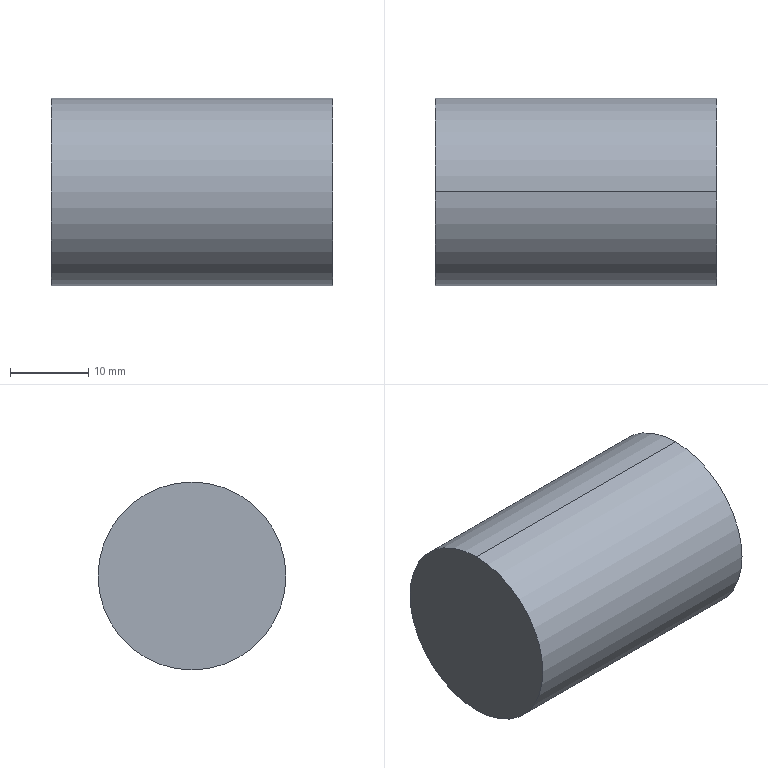Component | SolidWorks | PushRodCylinder-1 | 1 solid | 7 faces | box 36 x 24 x 24 mm | volume 15281 mm3 | cylinder 4 | plane 3 | commonest cylinder face diameters 8 x2 24 x2
build123d program:
from build123d import *

# Parameters (mm, degrees)
SKETCH1_R           = 12
BOSS_EXTRUDE1_DEPTH = 36
SKETCH2_R           = 4
CUT_EXTRUDE1_DEPTH  = 20


with BuildPart() as part:
    # Sketch1 → Boss-Extrude1 (new body)
    with BuildSketch(Plane.XY):
        Circle(SKETCH1_R)
    extrude(amount=BOSS_EXTRUDE1_DEPTH)

    # Sketch2 → Cut-Extrude1 (cut)
    with BuildSketch(Plane(origin=(0, 0, 0), x_dir=(-1, 0, 0), z_dir=(0, 0, -1))):
        Circle(SKETCH2_R)
    extrude(amount=-CUT_EXTRUDE1_DEPTH, mode=Mode.SUBTRACT)


solid = part.part

# Placed as in the assembly
solid = solid.moved(Location((-183.5, 220, -10), (0, -90, 0)))
STEP:
#1=COLOUR_RGB('',0.7922,0.8196,0.9333);
#2=FILL_AREA_STYLE_COLOUR('',#1);
#3=FILL_AREA_STYLE('',(#2));
#4=SURFACE_STYLE_FILL_AREA(#3);
#5=SURFACE_SIDE_STYLE('',(#4));
#6=SURFACE_STYLE_USAGE(.BOTH.,#5);
#7=PRESENTATION_STYLE_ASSIGNMENT((#6));
#8=CARTESIAN_POINT('',(-8.012,8.661,-0.2362));
#9=VERTEX_POINT('',#8);
#10=CARTESIAN_POINT('',(-8.012,8.661,-0.5512));
#11=VERTEX_POINT('',#10);
#12=CARTESIAN_POINT('',(-8.012,8.661,-0.3937));
#13=DIRECTION('',(1.,0.,0.));
#14=DIRECTION('',(0.,0.,-1.));
#15=AXIS2_PLACEMENT_3D('',#12,#13,#14);
#16=CIRCLE('',#15,0.1575);
#17=EDGE_CURVE('',#9,#11,#16,.T.);
#18=ORIENTED_EDGE('',*,*,#17,.F.);
#19=CARTESIAN_POINT('',(-7.224,8.661,-0.2362));
#20=VERTEX_POINT('',#19);
#21=CARTESIAN_POINT('',(-8.012,8.661,-0.2362));
#22=DIRECTION('',(1.,0.,0.));
#23=VECTOR('',#22,39.37);
#24=LINE('',#21,#23);
#25=EDGE_CURVE('',#9,#20,#24,.T.);
#26=ORIENTED_EDGE('',*,*,#25,.T.);
#27=CARTESIAN_POINT('',(-7.224,8.661,-0.5512));
#28=VERTEX_POINT('',#27);
#29=CARTESIAN_POINT('',(-7.224,8.661,-0.3937));
#30=DIRECTION('',(1.,0.,0.));
#31=DIRECTION('',(0.,0.,-1.));
#32=AXIS2_PLACEMENT_3D('',#29,#30,#31);
#33=CIRCLE('',#32,0.1575);
#34=EDGE_CURVE('',#20,#28,#33,.T.);
#35=ORIENTED_EDGE('',*,*,#34,.T.);
#36=CARTESIAN_POINT('',(-8.012,8.661,-0.5512));
#37=DIRECTION('',(1.,0.,0.));
#38=VECTOR('',#37,39.37);
#39=LINE('',#36,#38);
#40=EDGE_CURVE('',#11,#28,#39,.T.);
#41=ORIENTED_EDGE('',*,*,#40,.F.);
#42=EDGE_LOOP('',(#18,#26,#35,#41));
#43=FACE_OUTER_BOUND('',#42,.T.);
#44=CARTESIAN_POINT('',(-8.012,8.661,-0.3937));
#45=DIRECTION('',(1.,0.,0.));
#46=DIRECTION('',(0.,0.,-1.));
#47=AXIS2_PLACEMENT_3D('',#44,#45,#46);
#48=CYLINDRICAL_SURFACE('',#47,0.1575);
#49=ADVANCED_FACE('',(#43),#48,.F.);
#50=CARTESIAN_POINT('',(-8.642,8.661,0.07874));
#51=VERTEX_POINT('',#50);
#52=CARTESIAN_POINT('',(-8.642,8.661,-0.8661));
#53=VERTEX_POINT('',#52);
#54=CARTESIAN_POINT('',(-8.642,8.661,-0.3937));
#55=DIRECTION('',(-1.,0.,0.));
#56=DIRECTION('',(0.,0.,1.));
#57=AXIS2_PLACEMENT_3D('',#54,#55,#56);
#58=CIRCLE('',#57,0.4724);
#59=EDGE_CURVE('',#51,#53,#58,.T.);
#60=ORIENTED_EDGE('',*,*,#59,.F.);
#61=CARTESIAN_POINT('',(-7.224,8.661,0.07874));
#62=VERTEX_POINT('',#61);
#63=CARTESIAN_POINT('',(-8.642,8.661,0.07874));
#64=DIRECTION('',(1.,0.,0.));
#65=VECTOR('',#64,39.37);
#66=LINE('',#63,#65);
#67=EDGE_CURVE('',#51,#62,#66,.T.);
#68=ORIENTED_EDGE('',*,*,#67,.T.);
#69=CARTESIAN_POINT('',(-7.224,8.661,-0.8661));
#70=VERTEX_POINT('',#69);
#71=CARTESIAN_POINT('',(-7.224,8.661,-0.3937));
#72=DIRECTION('',(-1.,0.,0.));
#73=DIRECTION('',(0.,0.,1.));
#74=AXIS2_PLACEMENT_3D('',#71,#72,#73);
#75=CIRCLE('',#74,0.4724);
#76=EDGE_CURVE('',#62,#70,#75,.T.);
#77=ORIENTED_EDGE('',*,*,#76,.T.);
#78=CARTESIAN_POINT('',(-8.642,8.661,-0.8661));
#79=DIRECTION('',(1.,0.,0.));
#80=VECTOR('',#79,39.37);
#81=LINE('',#78,#80);
#82=EDGE_CURVE('',#53,#70,#81,.T.);
#83=ORIENTED_EDGE('',*,*,#82,.F.);
#84=EDGE_LOOP('',(#60,#68,#77,#83));
#85=FACE_OUTER_BOUND('',#84,.T.);
#86=CARTESIAN_POINT('',(-8.642,8.661,-0.3937));
#87=DIRECTION('',(1.,0.,0.));
#88=DIRECTION('',(0.,0.,-1.));
#89=AXIS2_PLACEMENT_3D('',#86,#87,#88);
#90=CYLINDRICAL_SURFACE('',#89,0.4724);
#91=ADVANCED_FACE('',(#85),#90,.T.);
#92=ORIENTED_EDGE('',*,*,#67,.F.);
#93=CARTESIAN_POINT('',(-8.642,8.661,-0.3937));
#94=DIRECTION('',(-1.,0.,0.));
#95=DIRECTION('',(0.,0.,1.));
#96=AXIS2_PLACEMENT_3D('',#93,#94,#95);
#97=CIRCLE('',#96,0.4724);
#98=EDGE_CURVE('',#53,#51,#97,.T.);
#99=ORIENTED_EDGE('',*,*,#98,.F.);
#100=ORIENTED_EDGE('',*,*,#82,.T.);
#101=CARTESIAN_POINT('',(-7.224,8.661,-0.3937));
#102=DIRECTION('',(-1.,0.,0.));
#103=DIRECTION('',(0.,0.,1.));
#104=AXIS2_PLACEMENT_3D('',#101,#102,#103);
#105=CIRCLE('',#104,0.4724);
#106=EDGE_CURVE('',#70,#62,#105,.T.);
#107=ORIENTED_EDGE('',*,*,#106,.T.);
#108=EDGE_LOOP('',(#92,#99,#100,#107));
#109=FACE_OUTER_BOUND('',#108,.T.);
#110=CARTESIAN_POINT('',(-8.642,8.661,-0.3937));
#111=DIRECTION('',(1.,0.,0.));
#112=DIRECTION('',(0.,0.,-1.));
#113=AXIS2_PLACEMENT_3D('',#110,#111,#112);
#114=CYLINDRICAL_SURFACE('',#113,0.4724);
#115=ADVANCED_FACE('',(#109),#114,.T.);
#116=ORIENTED_EDGE('',*,*,#98,.T.);
#117=ORIENTED_EDGE('',*,*,#59,.T.);
#118=EDGE_LOOP('',(#116,#117));
#119=FACE_OUTER_BOUND('',#118,.T.);
#120=CARTESIAN_POINT('',(-8.642,8.661,-0.3937));
#121=DIRECTION('',(-1.,0.,0.));
#122=DIRECTION('',(0.,0.,1.));
#123=AXIS2_PLACEMENT_3D('',#120,#121,#122);
#124=PLANE('',#123);
#125=ADVANCED_FACE('',(#119),#124,.T.);
#126=CARTESIAN_POINT('',(-7.224,8.661,-0.3937));
#127=DIRECTION('',(1.,0.,0.));
#128=DIRECTION('',(0.,0.,-1.));
#129=AXIS2_PLACEMENT_3D('',#126,#127,#128);
#130=CIRCLE('',#129,0.1575);
#131=EDGE_CURVE('',#28,#20,#130,.T.);
#132=ORIENTED_EDGE('',*,*,#131,.F.);
#133=ORIENTED_EDGE('',*,*,#34,.F.);
#134=EDGE_LOOP('',(#132,#133));
#135=FACE_BOUND('',#134,.T.);
#136=ORIENTED_EDGE('',*,*,#106,.F.);
#137=ORIENTED_EDGE('',*,*,#76,.F.);
#138=EDGE_LOOP('',(#136,#137));
#139=FACE_OUTER_BOUND('',#138,.T.);
#140=CARTESIAN_POINT('',(-7.224,8.661,-0.3937));
#141=DIRECTION('',(-1.,0.,0.));
#142=DIRECTION('',(0.,0.,1.));
#143=AXIS2_PLACEMENT_3D('',#140,#141,#142);
#144=PLANE('',#143);
#145=ADVANCED_FACE('',(#135,#139),#144,.F.);
#146=ORIENTED_EDGE('',*,*,#25,.F.);
#147=CARTESIAN_POINT('',(-8.012,8.661,-0.3937));
#148=DIRECTION('',(1.,0.,0.));
#149=DIRECTION('',(0.,0.,-1.));
#150=AXIS2_PLACEMENT_3D('',#147,#148,#149);
#151=CIRCLE('',#150,0.1575);
#152=EDGE_CURVE('',#11,#9,#151,.T.);
#153=ORIENTED_EDGE('',*,*,#152,.F.);
#154=ORIENTED_EDGE('',*,*,#40,.T.);
#155=ORIENTED_EDGE('',*,*,#131,.T.);
#156=EDGE_LOOP('',(#146,#153,#154,#155));
#157=FACE_OUTER_BOUND('',#156,.T.);
#158=CARTESIAN_POINT('',(-8.012,8.661,-0.3937));
#159=DIRECTION('',(1.,0.,0.));
#160=DIRECTION('',(0.,0.,-1.));
#161=AXIS2_PLACEMENT_3D('',#158,#159,#160);
#162=CYLINDRICAL_SURFACE('',#161,0.1575);
#163=ADVANCED_FACE('',(#157),#162,.F.);
#164=ORIENTED_EDGE('',*,*,#152,.T.);
#165=ORIENTED_EDGE('',*,*,#17,.T.);
#166=EDGE_LOOP('',(#164,#165));
#167=FACE_OUTER_BOUND('',#166,.T.);
#168=CARTESIAN_POINT('',(-8.012,8.661,-0.3937));
#169=DIRECTION('',(1.,0.,0.));
#170=DIRECTION('',(0.,0.,-1.));
#171=AXIS2_PLACEMENT_3D('',#168,#169,#170);
#172=PLANE('',#171);
#173=ADVANCED_FACE('',(#167),#172,.T.);
#174=CLOSED_SHELL('',(#49,#91,#115,#125,#145,#163,#173));
#175=MANIFOLD_SOLID_BREP('',#174);
#176=STYLED_ITEM('',(#7),#175);
#177=PRESENTATION_LAYER_ASSIGNMENT('','',(#176));
#178=CARTESIAN_POINT('',(0.,0.,0.));
#179=DIRECTION('',(0.,0.,1.));
#180=DIRECTION('',(1.,0.,0.));
#181=AXIS2_PLACEMENT_3D('',#178,#179,#180);
#182=(LENGTH_UNIT()NAMED_UNIT(*)SI_UNIT($,.METRE.));
#183=LENGTH_MEASURE_WITH_UNIT(LENGTH_MEASURE(0.0254),#182);
#184=DIMENSIONAL_EXPONENTS(1.,0.,0.,0.,0.,0.,0.);
#185=(CONVERSION_BASED_UNIT('',#183)LENGTH_UNIT()NAMED_UNIT(#184));
#186=UNCERTAINTY_MEASURE_WITH_UNIT(LENGTH_MEASURE(0.00001),#185,'','');
#187=(NAMED_UNIT(*)PLANE_ANGLE_UNIT()SI_UNIT($,.RADIAN.));
#188=(NAMED_UNIT(*)SI_UNIT($,.STERADIAN.)SOLID_ANGLE_UNIT());
#189=(GEOMETRIC_REPRESENTATION_CONTEXT(3)GLOBAL_UNCERTAINTY_ASSIGNED_CONTEXT((#186))GLOBAL_UNIT_ASSIGNED_CONTEXT((#185,#187,#188))REPRESENTATION_CONTEXT('',''));
#190=ADVANCED_BREP_SHAPE_REPRESENTATION('',(#175,#181),#189);
#191=(LENGTH_UNIT()NAMED_UNIT(*)SI_UNIT($,.METRE.));
#192=LENGTH_MEASURE_WITH_UNIT(LENGTH_MEASURE(0.0254),#191);
#193=DIMENSIONAL_EXPONENTS(1.,0.,0.,0.,0.,0.,0.);
#194=(CONVERSION_BASED_UNIT('',#192)LENGTH_UNIT()NAMED_UNIT(#193));
#195=UNCERTAINTY_MEASURE_WITH_UNIT(LENGTH_MEASURE(0.00001),#194,'','');
#196=(NAMED_UNIT(*)PLANE_ANGLE_UNIT()SI_UNIT($,.RADIAN.));
#197=(NAMED_UNIT(*)SI_UNIT($,.STERADIAN.)SOLID_ANGLE_UNIT());
#198=(GEOMETRIC_REPRESENTATION_CONTEXT(3)GLOBAL_UNCERTAINTY_ASSIGNED_CONTEXT((#195))GLOBAL_UNIT_ASSIGNED_CONTEXT((#194,#196,#197))REPRESENTATION_CONTEXT('',''));
#199=MECHANICAL_DESIGN_GEOMETRIC_PRESENTATION_REPRESENTATION('',(#176),#198);